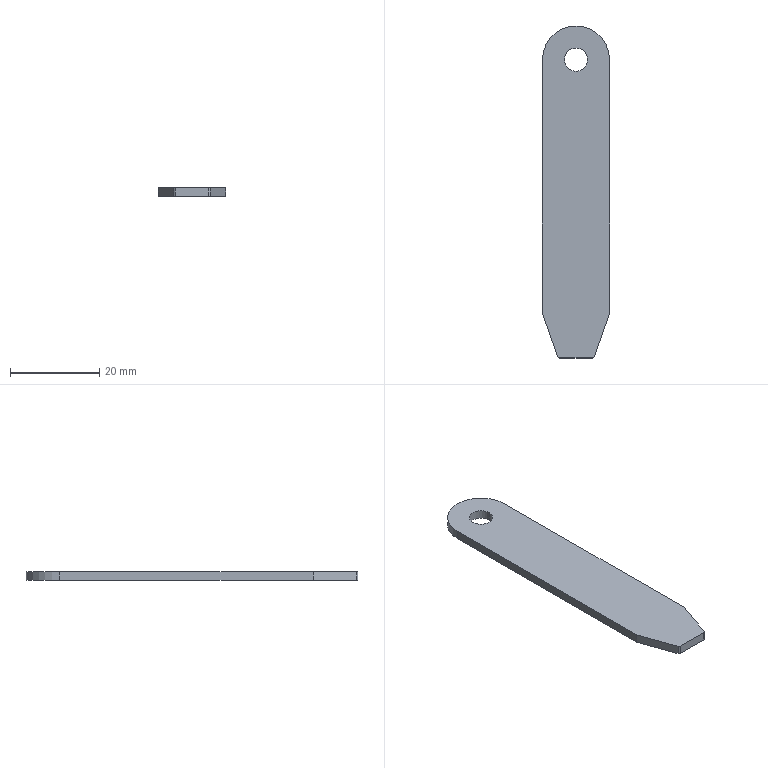Component | SolidWorks | CLS-MechanismTopPlate-1 | 1 solid | 13 faces | box 15 x 74.2 x 2 mm | volume 2065 mm3 | plane 7 | cylinder 6 | commonest cylinder face diameters 5.2 x2 15 x2 1 x2 | material 2.0 Galvanized Sheet Q235A
STEP:
#1=CARTESIAN_POINT('',(0.5147,-1.036,-0.1969));
#2=VERTEX_POINT('',#1);
#3=CARTESIAN_POINT('',(0.31,-1.036,-0.1969));
#4=VERTEX_POINT('',#3);
#5=CARTESIAN_POINT('',(0.4124,-1.036,-0.1969));
#6=DIRECTION('',(0.,0.,-1.));
#7=DIRECTION('',(-1.,0.,0.));
#8=AXIS2_PLACEMENT_3D('',#5,#6,#7);
#9=CIRCLE('',#8,0.1024);
#10=EDGE_CURVE('',#2,#4,#9,.T.);
#11=ORIENTED_EDGE('',*,*,#10,.F.);
#12=CARTESIAN_POINT('',(0.5147,-1.036,-0.2756));
#13=VERTEX_POINT('',#12);
#14=CARTESIAN_POINT('',(0.5147,-1.036,0.1181));
#15=DIRECTION('',(0.,0.,-1.));
#16=VECTOR('',#15,39.37);
#17=LINE('',#14,#16);
#18=EDGE_CURVE('',#2,#13,#17,.T.);
#19=ORIENTED_EDGE('',*,*,#18,.T.);
#20=CARTESIAN_POINT('',(0.31,-1.036,-0.2756));
#21=VERTEX_POINT('',#20);
#22=CARTESIAN_POINT('',(0.4124,-1.036,-0.2756));
#23=DIRECTION('',(0.,0.,-1.));
#24=DIRECTION('',(-1.,0.,0.));
#25=AXIS2_PLACEMENT_3D('',#22,#23,#24);
#26=CIRCLE('',#25,0.1024);
#27=EDGE_CURVE('',#13,#21,#26,.T.);
#28=ORIENTED_EDGE('',*,*,#27,.T.);
#29=CARTESIAN_POINT('',(0.31,-1.036,0.1181));
#30=DIRECTION('',(0.,0.,-1.));
#31=VECTOR('',#30,39.37);
#32=LINE('',#29,#31);
#33=EDGE_CURVE('',#4,#21,#32,.T.);
#34=ORIENTED_EDGE('',*,*,#33,.F.);
#35=EDGE_LOOP('',(#11,#19,#28,#34));
#36=FACE_OUTER_BOUND('',#35,.T.);
#37=CARTESIAN_POINT('',(0.4124,-1.036,0.1181));
#38=DIRECTION('',(0.,0.,-1.));
#39=DIRECTION('',(-1.,0.,0.));
#40=AXIS2_PLACEMENT_3D('',#37,#38,#39);
#41=CYLINDRICAL_SURFACE('',#40,0.1024);
#42=ADVANCED_FACE('',(#36),#41,.F.);
#43=CARTESIAN_POINT('',(0.1171,-1.036,-0.2756));
#44=VERTEX_POINT('',#43);
#45=CARTESIAN_POINT('',(0.1171,-3.268,-0.2756));
#46=VERTEX_POINT('',#45);
#47=CARTESIAN_POINT('',(0.1171,-0.7405,-0.2756));
#48=DIRECTION('',(0.,-1.,0.));
#49=VECTOR('',#48,39.37);
#50=LINE('',#47,#49);
#51=EDGE_CURVE('',#44,#46,#50,.T.);
#52=ORIENTED_EDGE('',*,*,#51,.T.);
#53=CARTESIAN_POINT('',(0.1171,-3.268,-0.1969));
#54=VERTEX_POINT('',#53);
#55=CARTESIAN_POINT('',(0.1171,-3.268,-0.2756));
#56=DIRECTION('',(0.,0.,1.));
#57=VECTOR('',#56,39.37);
#58=LINE('',#55,#57);
#59=EDGE_CURVE('',#46,#54,#58,.T.);
#60=ORIENTED_EDGE('',*,*,#59,.T.);
#61=CARTESIAN_POINT('',(0.1171,-1.036,-0.1969));
#62=VERTEX_POINT('',#61);
#63=CARTESIAN_POINT('',(0.1171,-0.7405,-0.1969));
#64=DIRECTION('',(0.,-1.,0.));
#65=VECTOR('',#64,39.37);
#66=LINE('',#63,#65);
#67=EDGE_CURVE('',#62,#54,#66,.T.);
#68=ORIENTED_EDGE('',*,*,#67,.F.);
#69=CARTESIAN_POINT('',(0.1171,-1.036,-0.2756));
#70=DIRECTION('',(0.,0.,-1.));
#71=VECTOR('',#70,39.37);
#72=LINE('',#69,#71);
#73=EDGE_CURVE('',#62,#44,#72,.T.);
#74=ORIENTED_EDGE('',*,*,#73,.T.);
#75=EDGE_LOOP('',(#52,#60,#68,#74));
#76=FACE_OUTER_BOUND('',#75,.T.);
#77=CARTESIAN_POINT('',(0.1171,-0.7405,-0.2756));
#78=DIRECTION('',(-1.,-0.,0.));
#79=DIRECTION('',(0.,-1.,0.));
#80=AXIS2_PLACEMENT_3D('',#77,#78,#79);
#81=PLANE('',#80);
#82=ADVANCED_FACE('',(#76),#81,.T.);
#83=CARTESIAN_POINT('',(0.7076,-3.268,-0.1969));
#84=VERTEX_POINT('',#83);
#85=CARTESIAN_POINT('',(0.7076,-1.036,-0.1969));
#86=VERTEX_POINT('',#85);
#87=CARTESIAN_POINT('',(0.7076,-0.7405,-0.1969));
#88=DIRECTION('',(-0.,1.,0.));
#89=VECTOR('',#88,39.37);
#90=LINE('',#87,#89);
#91=EDGE_CURVE('',#84,#86,#90,.T.);
#92=ORIENTED_EDGE('',*,*,#91,.F.);
#93=CARTESIAN_POINT('',(0.7076,-3.268,-0.2756));
#94=VERTEX_POINT('',#93);
#95=CARTESIAN_POINT('',(0.7076,-3.268,-0.2756));
#96=DIRECTION('',(0.,0.,-1.));
#97=VECTOR('',#96,39.37);
#98=LINE('',#95,#97);
#99=EDGE_CURVE('',#84,#94,#98,.T.);
#100=ORIENTED_EDGE('',*,*,#99,.T.);
#101=CARTESIAN_POINT('',(0.7076,-1.036,-0.2756));
#102=VERTEX_POINT('',#101);
#103=CARTESIAN_POINT('',(0.7076,-0.7405,-0.2756));
#104=DIRECTION('',(-0.,1.,0.));
#105=VECTOR('',#104,39.37);
#106=LINE('',#103,#105);
#107=EDGE_CURVE('',#94,#102,#106,.T.);
#108=ORIENTED_EDGE('',*,*,#107,.T.);
#109=CARTESIAN_POINT('',(0.7076,-1.036,-0.2756));
#110=DIRECTION('',(0.,0.,1.));
#111=VECTOR('',#110,39.37);
#112=LINE('',#109,#111);
#113=EDGE_CURVE('',#102,#86,#112,.T.);
#114=ORIENTED_EDGE('',*,*,#113,.T.);
#115=EDGE_LOOP('',(#92,#100,#108,#114));
#116=FACE_OUTER_BOUND('',#115,.T.);
#117=CARTESIAN_POINT('',(0.7076,-0.7405,-0.2756));
#118=DIRECTION('',(1.,0.,0.));
#119=DIRECTION('',(-0.,1.,0.));
#120=AXIS2_PLACEMENT_3D('',#117,#118,#119);
#121=PLANE('',#120);
#122=ADVANCED_FACE('',(#116),#121,.T.);
#123=CARTESIAN_POINT('',(0.2688,-3.662,-0.2756));
#124=VERTEX_POINT('',#123);
#125=CARTESIAN_POINT('',(0.5559,-3.662,-0.2756));
#126=VERTEX_POINT('',#125);
#127=CARTESIAN_POINT('',(0.7076,-3.662,-0.2756));
#128=DIRECTION('',(1.,0.,0.));
#129=VECTOR('',#128,39.37);
#130=LINE('',#127,#129);
#131=EDGE_CURVE('',#124,#126,#130,.T.);
#132=ORIENTED_EDGE('',*,*,#131,.T.);
#133=CARTESIAN_POINT('',(0.5559,-3.662,-0.1969));
#134=VERTEX_POINT('',#133);
#135=CARTESIAN_POINT('',(0.5559,-3.662,-0.2756));
#136=DIRECTION('',(0.,0.,1.));
#137=VECTOR('',#136,39.37);
#138=LINE('',#135,#137);
#139=EDGE_CURVE('',#126,#134,#138,.T.);
#140=ORIENTED_EDGE('',*,*,#139,.T.);
#141=CARTESIAN_POINT('',(0.2688,-3.662,-0.1969));
#142=VERTEX_POINT('',#141);
#143=CARTESIAN_POINT('',(0.7076,-3.662,-0.1969));
#144=DIRECTION('',(1.,0.,0.));
#145=VECTOR('',#144,39.37);
#146=LINE('',#143,#145);
#147=EDGE_CURVE('',#142,#134,#146,.T.);
#148=ORIENTED_EDGE('',*,*,#147,.F.);
#149=CARTESIAN_POINT('',(0.2688,-3.662,-0.2756));
#150=DIRECTION('',(0.,0.,-1.));
#151=VECTOR('',#150,39.37);
#152=LINE('',#149,#151);
#153=EDGE_CURVE('',#142,#124,#152,.T.);
#154=ORIENTED_EDGE('',*,*,#153,.T.);
#155=EDGE_LOOP('',(#132,#140,#148,#154));
#156=FACE_OUTER_BOUND('',#155,.T.);
#157=CARTESIAN_POINT('',(0.7076,-3.662,-0.2756));
#158=DIRECTION('',(0.,-1.,0.));
#159=DIRECTION('',(0.,0.,-1.));
#160=AXIS2_PLACEMENT_3D('',#157,#158,#159);
#161=PLANE('',#160);
#162=ADVANCED_FACE('',(#156),#161,.T.);
#163=CARTESIAN_POINT('',(0.4124,-1.036,-0.2756));
#164=DIRECTION('',(0.,0.,-1.));
#165=DIRECTION('',(-1.,0.,0.));
#166=AXIS2_PLACEMENT_3D('',#163,#164,#165);
#167=CIRCLE('',#166,0.1024);
#168=EDGE_CURVE('',#21,#13,#167,.T.);
#169=ORIENTED_EDGE('',*,*,#168,.F.);
#170=ORIENTED_EDGE('',*,*,#27,.F.);
#171=EDGE_LOOP('',(#169,#170));
#172=FACE_BOUND('',#171,.T.);
#173=CARTESIAN_POINT('',(0.5744,-3.649,-0.2756));
#174=VERTEX_POINT('',#173);
#175=CARTESIAN_POINT('',(0.5204,-3.803,-0.2756));
#176=DIRECTION('',(-0.3304,-0.9439,0.));
#177=VECTOR('',#176,39.37);
#178=LINE('',#175,#177);
#179=EDGE_CURVE('',#94,#174,#178,.T.);
#180=ORIENTED_EDGE('',*,*,#179,.T.);
#181=CARTESIAN_POINT('',(0.5559,-3.642,-0.2756));
#182=DIRECTION('',(0.,0.,-1.));
#183=DIRECTION('',(-1.,0.,0.));
#184=AXIS2_PLACEMENT_3D('',#181,#182,#183);
#185=CIRCLE('',#184,0.01969);
#186=EDGE_CURVE('',#174,#126,#185,.T.);
#187=ORIENTED_EDGE('',*,*,#186,.T.);
#188=ORIENTED_EDGE('',*,*,#131,.F.);
#189=CARTESIAN_POINT('',(0.2503,-3.649,-0.2756));
#190=VERTEX_POINT('',#189);
#191=CARTESIAN_POINT('',(0.2688,-3.642,-0.2756));
#192=DIRECTION('',(0.,0.,-1.));
#193=DIRECTION('',(-1.,0.,0.));
#194=AXIS2_PLACEMENT_3D('',#191,#192,#193);
#195=CIRCLE('',#194,0.01969);
#196=EDGE_CURVE('',#124,#190,#195,.T.);
#197=ORIENTED_EDGE('',*,*,#196,.T.);
#198=CARTESIAN_POINT('',(0.2398,-3.619,-0.2756));
#199=DIRECTION('',(-0.3304,0.9439,0.));
#200=VECTOR('',#199,39.37);
#201=LINE('',#198,#200);
#202=EDGE_CURVE('',#190,#46,#201,.T.);
#203=ORIENTED_EDGE('',*,*,#202,.T.);
#204=ORIENTED_EDGE('',*,*,#51,.F.);
#205=CARTESIAN_POINT('',(0.4124,-0.7405,-0.2756));
#206=VERTEX_POINT('',#205);
#207=CARTESIAN_POINT('',(0.4124,-1.036,-0.2756));
#208=DIRECTION('',(0.,0.,-1.));
#209=DIRECTION('',(-1.,0.,0.));
#210=AXIS2_PLACEMENT_3D('',#207,#208,#209);
#211=CIRCLE('',#210,0.2953);
#212=EDGE_CURVE('',#44,#206,#211,.T.);
#213=ORIENTED_EDGE('',*,*,#212,.T.);
#214=CARTESIAN_POINT('',(0.4124,-1.036,-0.2756));
#215=DIRECTION('',(0.,0.,-1.));
#216=DIRECTION('',(-1.,0.,0.));
#217=AXIS2_PLACEMENT_3D('',#214,#215,#216);
#218=CIRCLE('',#217,0.2953);
#219=EDGE_CURVE('',#206,#102,#218,.T.);
#220=ORIENTED_EDGE('',*,*,#219,.T.);
#221=ORIENTED_EDGE('',*,*,#107,.F.);
#222=EDGE_LOOP('',(#180,#187,#188,#197,#203,#204,#213,#220,#221));
#223=FACE_OUTER_BOUND('',#222,.T.);
#224=CARTESIAN_POINT('',(0.1171,-3.662,-0.2756));
#225=DIRECTION('',(0.,0.,-1.));
#226=DIRECTION('',(-1.,0.,0.));
#227=AXIS2_PLACEMENT_3D('',#224,#225,#226);
#228=PLANE('',#227);
#229=ADVANCED_FACE('',(#172,#223),#228,.T.);
#230=CARTESIAN_POINT('',(0.4124,-1.036,-0.1969));
#231=DIRECTION('',(0.,0.,-1.));
#232=DIRECTION('',(-1.,0.,0.));
#233=AXIS2_PLACEMENT_3D('',#230,#231,#232);
#234=CIRCLE('',#233,0.1024);
#235=EDGE_CURVE('',#4,#2,#234,.T.);
#236=ORIENTED_EDGE('',*,*,#235,.T.);
#237=ORIENTED_EDGE('',*,*,#10,.T.);
#238=EDGE_LOOP('',(#236,#237));
#239=FACE_BOUND('',#238,.T.);
#240=ORIENTED_EDGE('',*,*,#147,.T.);
#241=CARTESIAN_POINT('',(0.5744,-3.649,-0.1969));
#242=VERTEX_POINT('',#241);
#243=CARTESIAN_POINT('',(0.5559,-3.642,-0.1969));
#244=DIRECTION('',(0.,0.,1.));
#245=DIRECTION('',(-1.,0.,0.));
#246=AXIS2_PLACEMENT_3D('',#243,#244,#245);
#247=CIRCLE('',#246,0.01969);
#248=EDGE_CURVE('',#134,#242,#247,.T.);
#249=ORIENTED_EDGE('',*,*,#248,.T.);
#250=CARTESIAN_POINT('',(0.5698,-3.662,-0.1969));
#251=DIRECTION('',(0.3304,0.9439,0.));
#252=VECTOR('',#251,39.37);
#253=LINE('',#250,#252);
#254=EDGE_CURVE('',#242,#84,#253,.T.);
#255=ORIENTED_EDGE('',*,*,#254,.T.);
#256=ORIENTED_EDGE('',*,*,#91,.T.);
#257=CARTESIAN_POINT('',(0.4124,-0.7405,-0.1969));
#258=VERTEX_POINT('',#257);
#259=CARTESIAN_POINT('',(0.4124,-1.036,-0.1969));
#260=DIRECTION('',(0.,0.,1.));
#261=DIRECTION('',(-1.,0.,0.));
#262=AXIS2_PLACEMENT_3D('',#259,#260,#261);
#263=CIRCLE('',#262,0.2953);
#264=EDGE_CURVE('',#86,#258,#263,.T.);
#265=ORIENTED_EDGE('',*,*,#264,.T.);
#266=CARTESIAN_POINT('',(0.4124,-1.036,-0.1969));
#267=DIRECTION('',(0.,0.,1.));
#268=DIRECTION('',(-1.,0.,0.));
#269=AXIS2_PLACEMENT_3D('',#266,#267,#268);
#270=CIRCLE('',#269,0.2953);
#271=EDGE_CURVE('',#258,#62,#270,.T.);
#272=ORIENTED_EDGE('',*,*,#271,.T.);
#273=ORIENTED_EDGE('',*,*,#67,.T.);
#274=CARTESIAN_POINT('',(0.2503,-3.649,-0.1969));
#275=VERTEX_POINT('',#274);
#276=CARTESIAN_POINT('',(0.1171,-3.268,-0.1969));
#277=DIRECTION('',(0.3304,-0.9439,0.));
#278=VECTOR('',#277,39.37);
#279=LINE('',#276,#278);
#280=EDGE_CURVE('',#54,#275,#279,.T.);
#281=ORIENTED_EDGE('',*,*,#280,.T.);
#282=CARTESIAN_POINT('',(0.2688,-3.642,-0.1969));
#283=DIRECTION('',(0.,0.,1.));
#284=DIRECTION('',(-1.,0.,0.));
#285=AXIS2_PLACEMENT_3D('',#282,#283,#284);
#286=CIRCLE('',#285,0.01969);
#287=EDGE_CURVE('',#275,#142,#286,.T.);
#288=ORIENTED_EDGE('',*,*,#287,.T.);
#289=EDGE_LOOP('',(#240,#249,#255,#256,#265,#272,#273,#281,#288));
#290=FACE_OUTER_BOUND('',#289,.T.);
#291=CARTESIAN_POINT('',(0.1171,-3.662,-0.1969));
#292=DIRECTION('',(0.,0.,-1.));
#293=DIRECTION('',(-1.,0.,0.));
#294=AXIS2_PLACEMENT_3D('',#291,#292,#293);
#295=PLANE('',#294);
#296=ADVANCED_FACE('',(#239,#290),#295,.F.);
#297=ORIENTED_EDGE('',*,*,#113,.F.);
#298=ORIENTED_EDGE('',*,*,#219,.F.);
#299=CARTESIAN_POINT('',(0.4124,-0.7405,-0.2756));
#300=DIRECTION('',(0.,0.,-1.));
#301=VECTOR('',#300,39.37);
#302=LINE('',#299,#301);
#303=EDGE_CURVE('',#258,#206,#302,.T.);
#304=ORIENTED_EDGE('',*,*,#303,.F.);
#305=ORIENTED_EDGE('',*,*,#264,.F.);
#306=EDGE_LOOP('',(#297,#298,#304,#305));
#307=FACE_OUTER_BOUND('',#306,.T.);
#308=CARTESIAN_POINT('',(0.4124,-1.036,-0.2756));
#309=DIRECTION('',(0.,0.,1.));
#310=DIRECTION('',(1.,0.,0.));
#311=AXIS2_PLACEMENT_3D('',#308,#309,#310);
#312=CYLINDRICAL_SURFACE('',#311,0.2953);
#313=ADVANCED_FACE('',(#307),#312,.T.);
#314=ORIENTED_EDGE('',*,*,#212,.F.);
#315=ORIENTED_EDGE('',*,*,#73,.F.);
#316=ORIENTED_EDGE('',*,*,#271,.F.);
#317=ORIENTED_EDGE('',*,*,#303,.T.);
#318=EDGE_LOOP('',(#314,#315,#316,#317));
#319=FACE_OUTER_BOUND('',#318,.T.);
#320=CARTESIAN_POINT('',(0.4124,-1.036,-0.2756));
#321=DIRECTION('',(0.,0.,1.));
#322=DIRECTION('',(1.,0.,0.));
#323=AXIS2_PLACEMENT_3D('',#320,#321,#322);
#324=CYLINDRICAL_SURFACE('',#323,0.2953);
#325=ADVANCED_FACE('',(#319),#324,.T.);
#326=ORIENTED_EDGE('',*,*,#18,.F.);
#327=ORIENTED_EDGE('',*,*,#235,.F.);
#328=ORIENTED_EDGE('',*,*,#33,.T.);
#329=ORIENTED_EDGE('',*,*,#168,.T.);
#330=EDGE_LOOP('',(#326,#327,#328,#329));
#331=FACE_OUTER_BOUND('',#330,.T.);
#332=CARTESIAN_POINT('',(0.4124,-1.036,0.1181));
#333=DIRECTION('',(0.,0.,-1.));
#334=DIRECTION('',(-1.,0.,0.));
#335=AXIS2_PLACEMENT_3D('',#332,#333,#334);
#336=CYLINDRICAL_SURFACE('',#335,0.1024);
#337=ADVANCED_FACE('',(#331),#336,.F.);
#338=ORIENTED_EDGE('',*,*,#202,.F.);
#339=CARTESIAN_POINT('',(0.2503,-3.649,-0.2756));
#340=DIRECTION('',(0.,0.,1.));
#341=VECTOR('',#340,39.37);
#342=LINE('',#339,#341);
#343=EDGE_CURVE('',#190,#275,#342,.T.);
#344=ORIENTED_EDGE('',*,*,#343,.T.);
#345=ORIENTED_EDGE('',*,*,#280,.F.);
#346=ORIENTED_EDGE('',*,*,#59,.F.);
#347=EDGE_LOOP('',(#338,#344,#345,#346));
#348=FACE_OUTER_BOUND('',#347,.T.);
#349=CARTESIAN_POINT('',(0.1171,-3.268,-0.2756));
#350=DIRECTION('',(0.9439,0.3304,0.));
#351=DIRECTION('',(-0.3304,0.9439,0.));
#352=AXIS2_PLACEMENT_3D('',#349,#350,#351);
#353=PLANE('',#352);
#354=ADVANCED_FACE('',(#348),#353,.F.);
#355=ORIENTED_EDGE('',*,*,#254,.F.);
#356=CARTESIAN_POINT('',(0.5744,-3.649,-0.2756));
#357=DIRECTION('',(0.,0.,-1.));
#358=VECTOR('',#357,39.37);
#359=LINE('',#356,#358);
#360=EDGE_CURVE('',#242,#174,#359,.T.);
#361=ORIENTED_EDGE('',*,*,#360,.T.);
#362=ORIENTED_EDGE('',*,*,#179,.F.);
#363=ORIENTED_EDGE('',*,*,#99,.F.);
#364=EDGE_LOOP('',(#355,#361,#362,#363));
#365=FACE_OUTER_BOUND('',#364,.T.);
#366=CARTESIAN_POINT('',(0.5698,-3.662,-0.2756));
#367=DIRECTION('',(-0.9439,0.3304,0.));
#368=DIRECTION('',(-0.3304,-0.9439,0.));
#369=AXIS2_PLACEMENT_3D('',#366,#367,#368);
#370=PLANE('',#369);
#371=ADVANCED_FACE('',(#365),#370,.F.);
#372=ORIENTED_EDGE('',*,*,#186,.F.);
#373=ORIENTED_EDGE('',*,*,#360,.F.);
#374=ORIENTED_EDGE('',*,*,#248,.F.);
#375=ORIENTED_EDGE('',*,*,#139,.F.);
#376=EDGE_LOOP('',(#372,#373,#374,#375));
#377=FACE_OUTER_BOUND('',#376,.T.);
#378=CARTESIAN_POINT('',(0.5559,-3.642,-0.2756));
#379=DIRECTION('',(0.,0.,-1.));
#380=DIRECTION('',(-1.,0.,0.));
#381=AXIS2_PLACEMENT_3D('',#378,#379,#380);
#382=CYLINDRICAL_SURFACE('',#381,0.01969);
#383=ADVANCED_FACE('',(#377),#382,.T.);
#384=ORIENTED_EDGE('',*,*,#287,.F.);
#385=ORIENTED_EDGE('',*,*,#343,.F.);
#386=ORIENTED_EDGE('',*,*,#196,.F.);
#387=ORIENTED_EDGE('',*,*,#153,.F.);
#388=EDGE_LOOP('',(#384,#385,#386,#387));
#389=FACE_OUTER_BOUND('',#388,.T.);
#390=CARTESIAN_POINT('',(0.2688,-3.642,-0.2756));
#391=DIRECTION('',(0.,0.,1.));
#392=DIRECTION('',(1.,0.,0.));
#393=AXIS2_PLACEMENT_3D('',#390,#391,#392);
#394=CYLINDRICAL_SURFACE('',#393,0.01969);
#395=ADVANCED_FACE('',(#389),#394,.T.);
#396=CLOSED_SHELL('',(#42,#82,#122,#162,#229,#296,#313,#325,#337,#354,#371,#383,#395));
#397=MANIFOLD_SOLID_BREP('',#396);
#398=CARTESIAN_POINT('',(0.,0.,0.));
#399=DIRECTION('',(0.,0.,1.));
#400=DIRECTION('',(1.,0.,0.));
#401=AXIS2_PLACEMENT_3D('',#398,#399,#400);
#402=(LENGTH_UNIT()NAMED_UNIT(*)SI_UNIT($,.METRE.));
#403=LENGTH_MEASURE_WITH_UNIT(LENGTH_MEASURE(0.0254),#402);
#404=DIMENSIONAL_EXPONENTS(1.,0.,0.,0.,0.,0.,0.);
#405=(CONVERSION_BASED_UNIT('',#403)LENGTH_UNIT()NAMED_UNIT(#404));
#406=UNCERTAINTY_MEASURE_WITH_UNIT(LENGTH_MEASURE(0.00001),#405,'','');
#407=(NAMED_UNIT(*)PLANE_ANGLE_UNIT()SI_UNIT($,.RADIAN.));
#408=(NAMED_UNIT(*)SI_UNIT($,.STERADIAN.)SOLID_ANGLE_UNIT());
#409=(GEOMETRIC_REPRESENTATION_CONTEXT(3)GLOBAL_UNCERTAINTY_ASSIGNED_CONTEXT((#406))GLOBAL_UNIT_ASSIGNED_CONTEXT((#405,#407,#408))REPRESENTATION_CONTEXT('',''));
#410=ADVANCED_BREP_SHAPE_REPRESENTATION('',(#397,#401),#409);
#411=COLOUR_RGB('',0.7922,0.8196,0.9333);
#412=FILL_AREA_STYLE_COLOUR('',#411);
#413=FILL_AREA_STYLE('',(#412));
#414=SURFACE_STYLE_FILL_AREA(#413);
#415=SURFACE_SIDE_STYLE('',(#414));
#416=SURFACE_STYLE_USAGE(.BOTH.,#415);
#417=PRESENTATION_STYLE_ASSIGNMENT((#416));
#418=STYLED_ITEM('',(#417),#397);
#419=(LENGTH_UNIT()NAMED_UNIT(*)SI_UNIT($,.METRE.));
#420=LENGTH_MEASURE_WITH_UNIT(LENGTH_MEASURE(0.0254),#419);
#421=DIMENSIONAL_EXPONENTS(1.,0.,0.,0.,0.,0.,0.);
#422=(CONVERSION_BASED_UNIT('',#420)LENGTH_UNIT()NAMED_UNIT(#421));
#423=UNCERTAINTY_MEASURE_WITH_UNIT(LENGTH_MEASURE(0.00001),#422,'','');
#424=(NAMED_UNIT(*)PLANE_ANGLE_UNIT()SI_UNIT($,.RADIAN.));
#425=(NAMED_UNIT(*)SI_UNIT($,.STERADIAN.)SOLID_ANGLE_UNIT());
#426=(GEOMETRIC_REPRESENTATION_CONTEXT(3)GLOBAL_UNCERTAINTY_ASSIGNED_CONTEXT((#423))GLOBAL_UNIT_ASSIGNED_CONTEXT((#422,#424,#425))REPRESENTATION_CONTEXT('',''));
#427=MECHANICAL_DESIGN_GEOMETRIC_PRESENTATION_REPRESENTATION('',(#418),#426);
#428=PRESENTATION_LAYER_ASSIGNMENT('','',(#418));